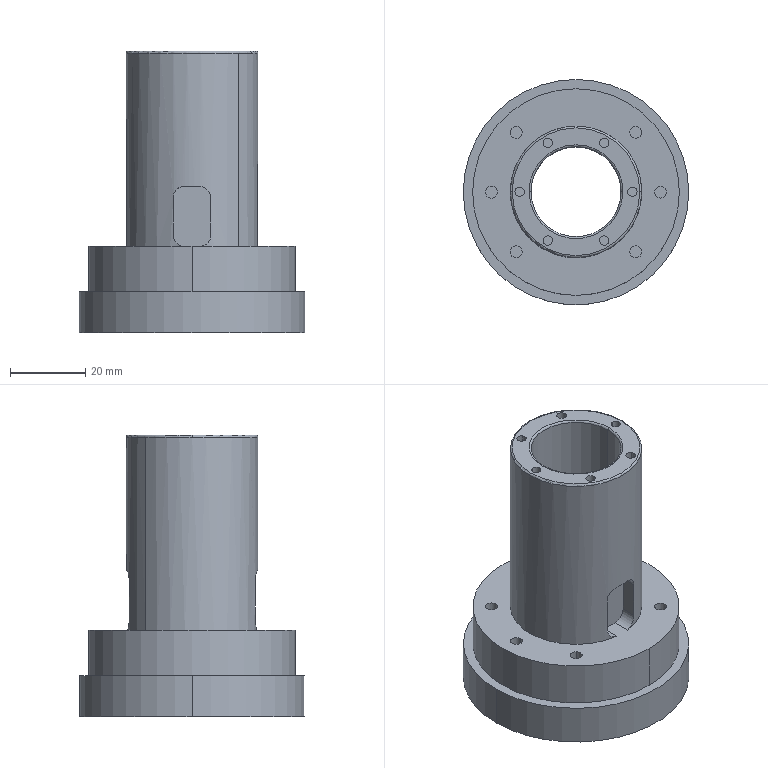CAM job | Mastercam | mm | 3 operations | part box 60 x 60 x 75
1. Drill/Counterbore | 17 - 6 倒角刀
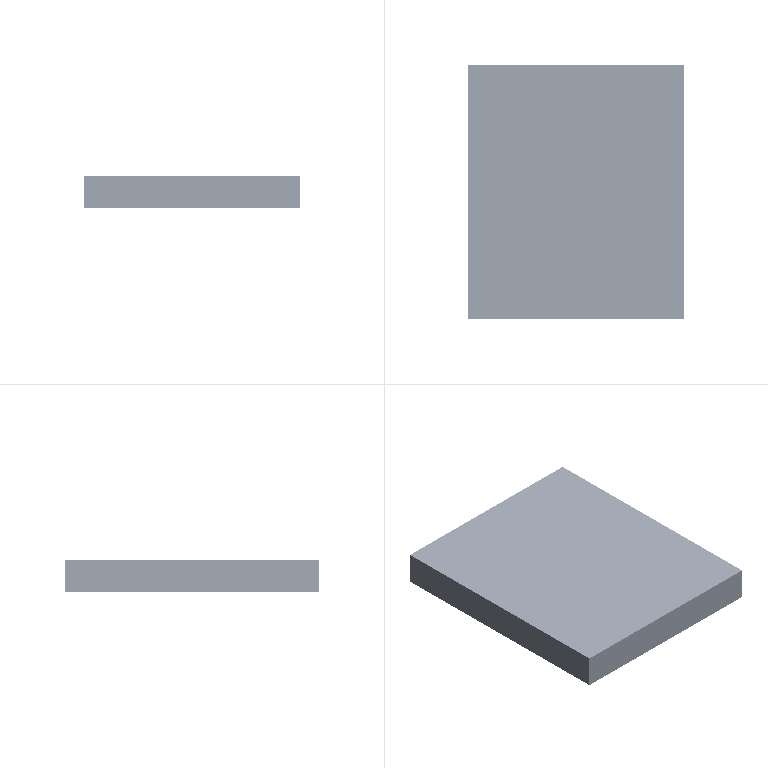2. 2D High Speed (2D Area Mill) | 4 - 4 平铣刀
3. Contour (Ramp) | 4 - 4 平铣刀